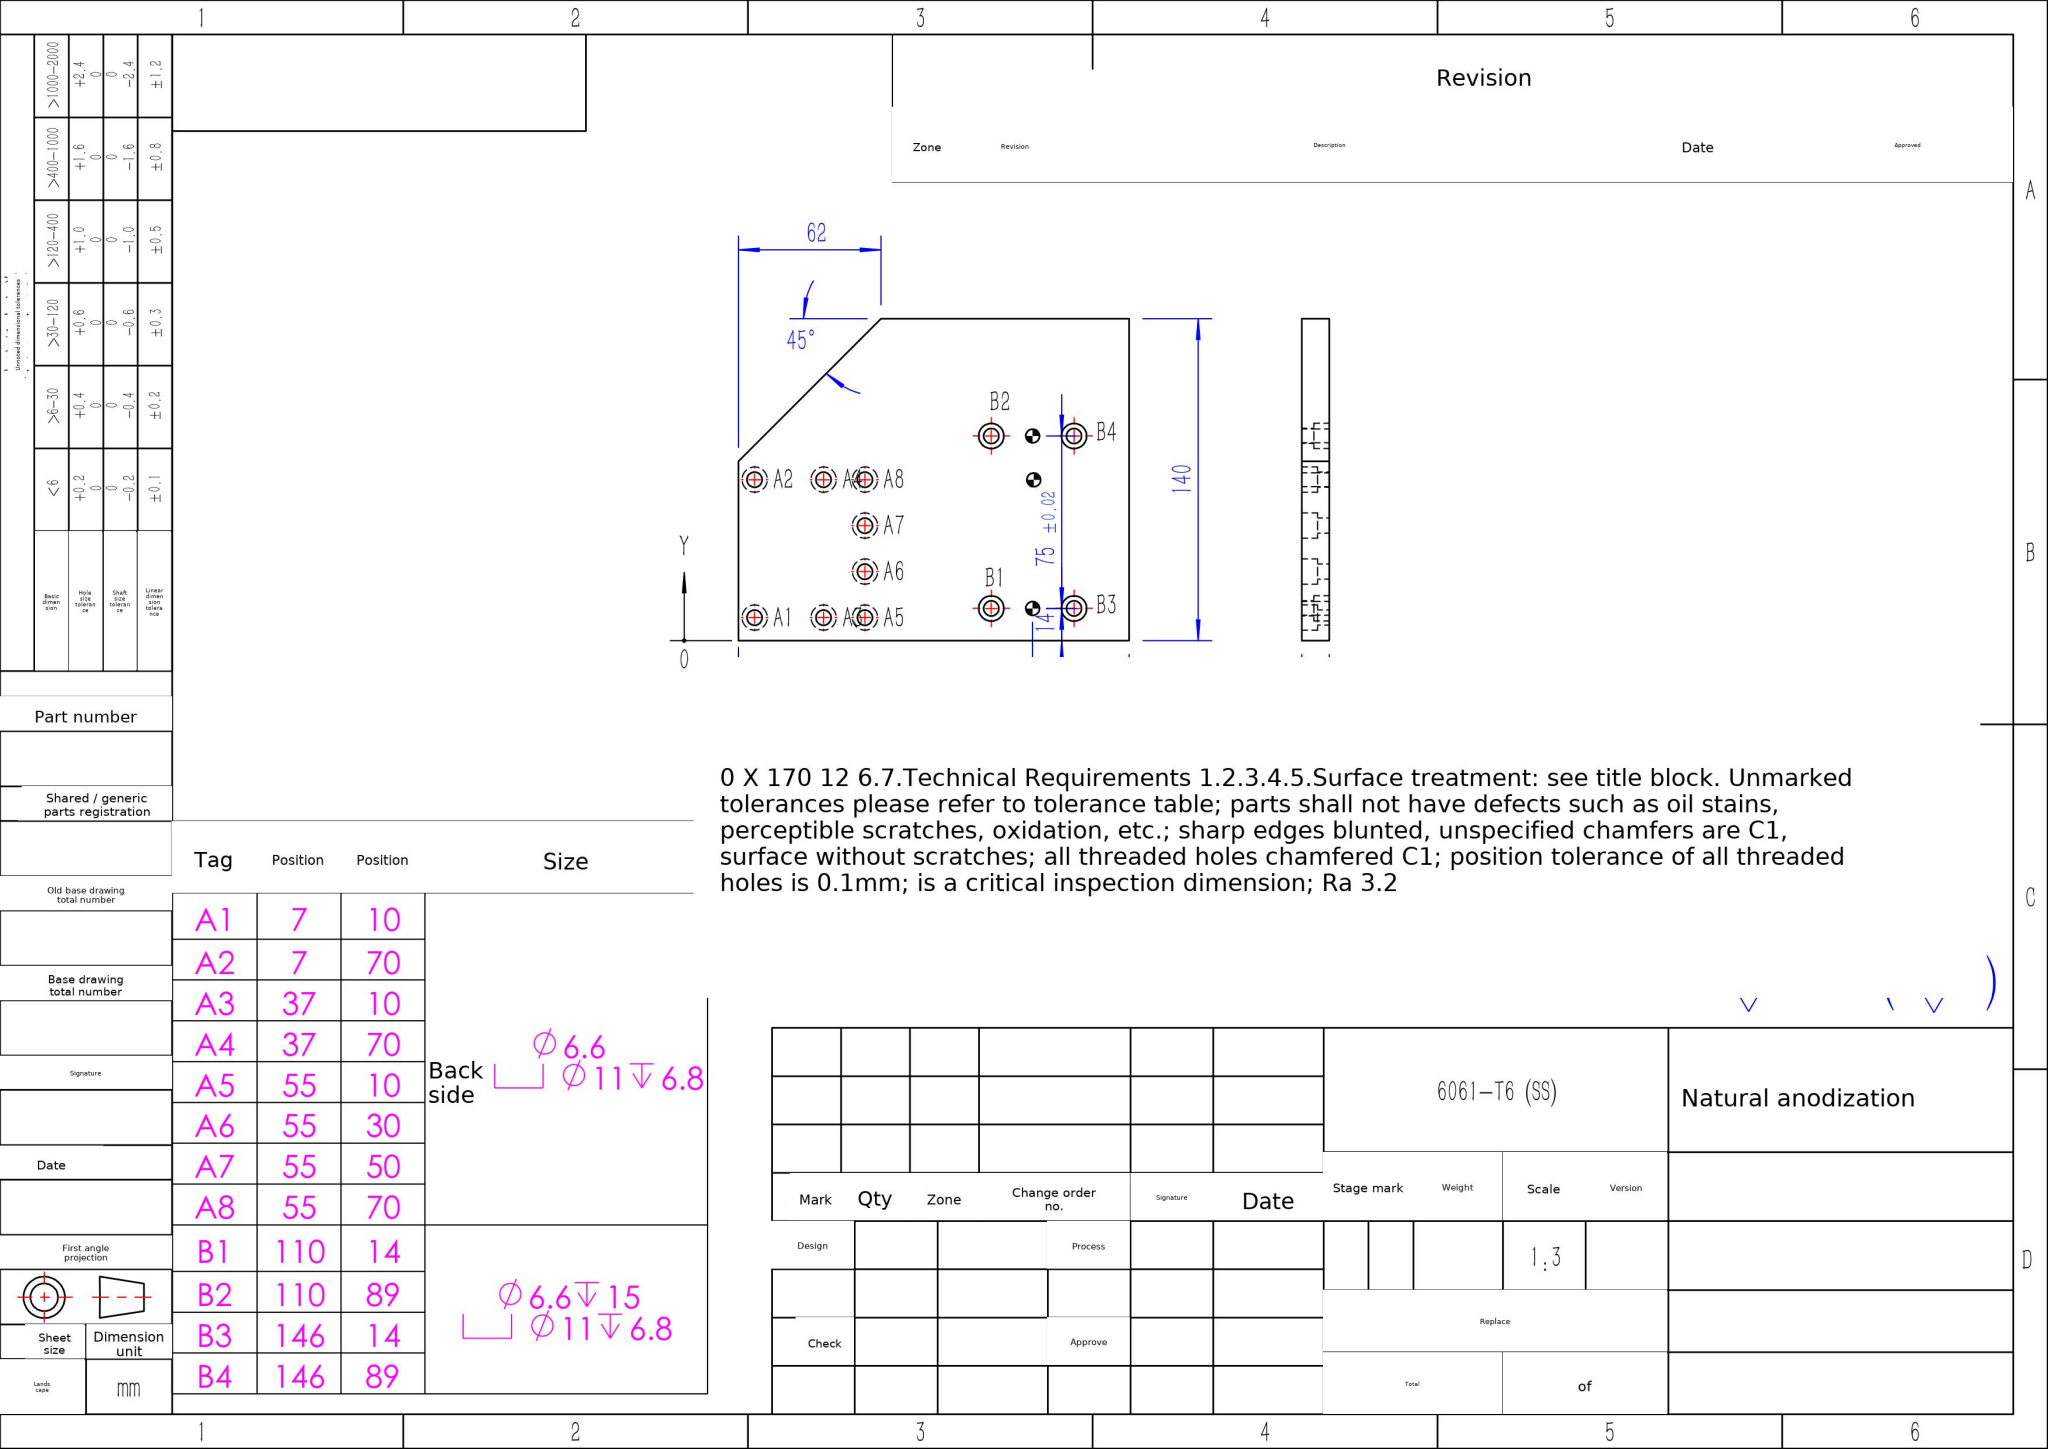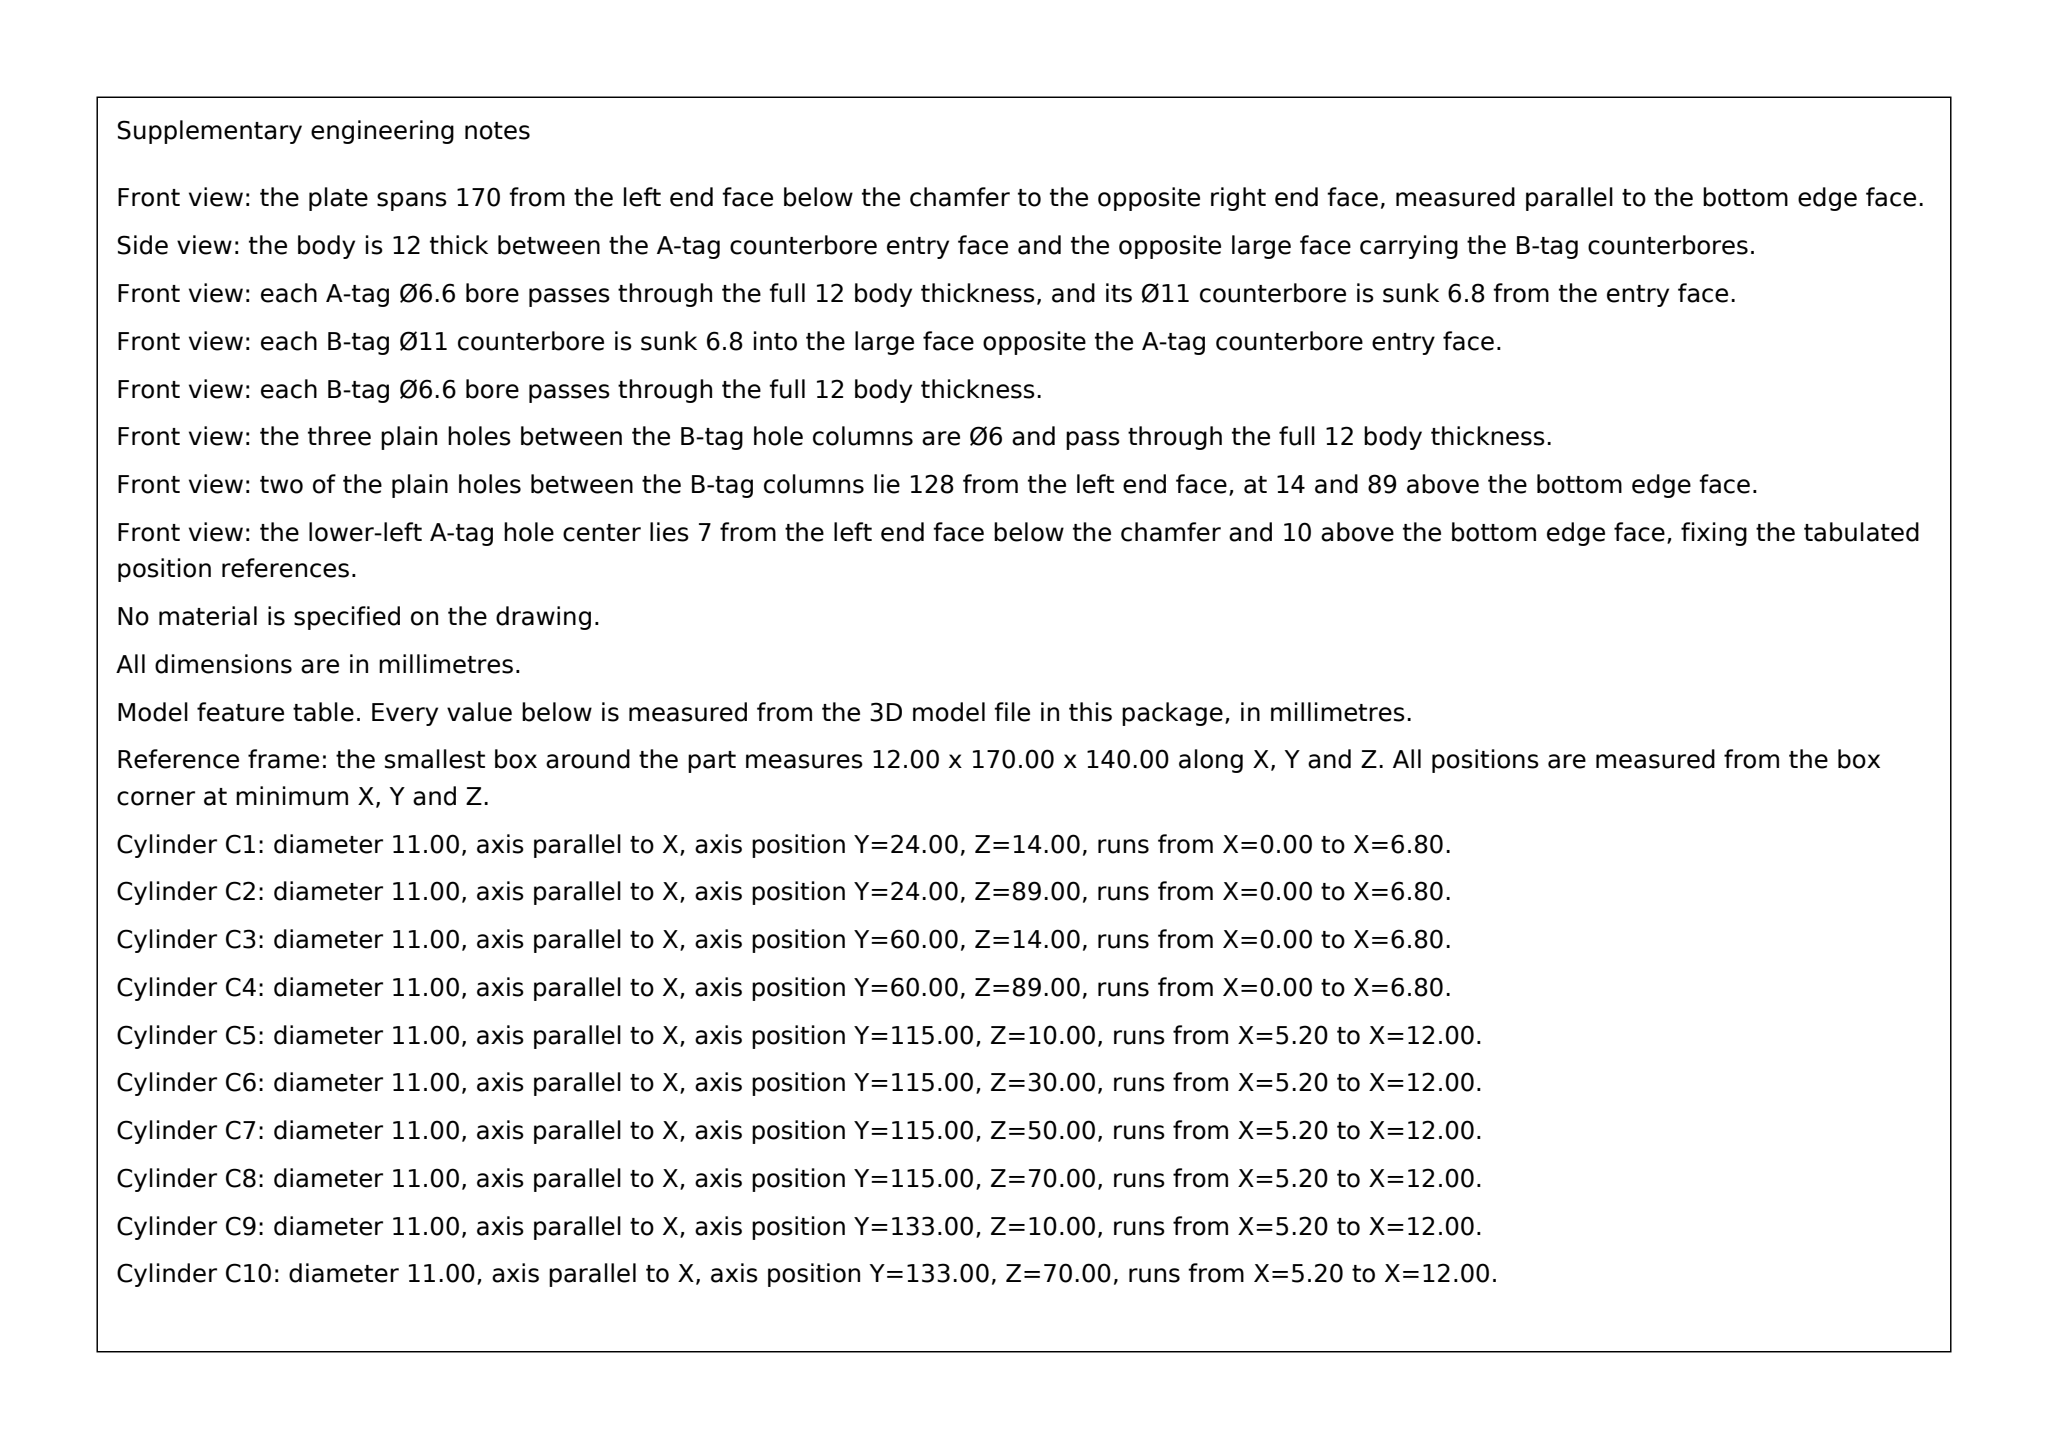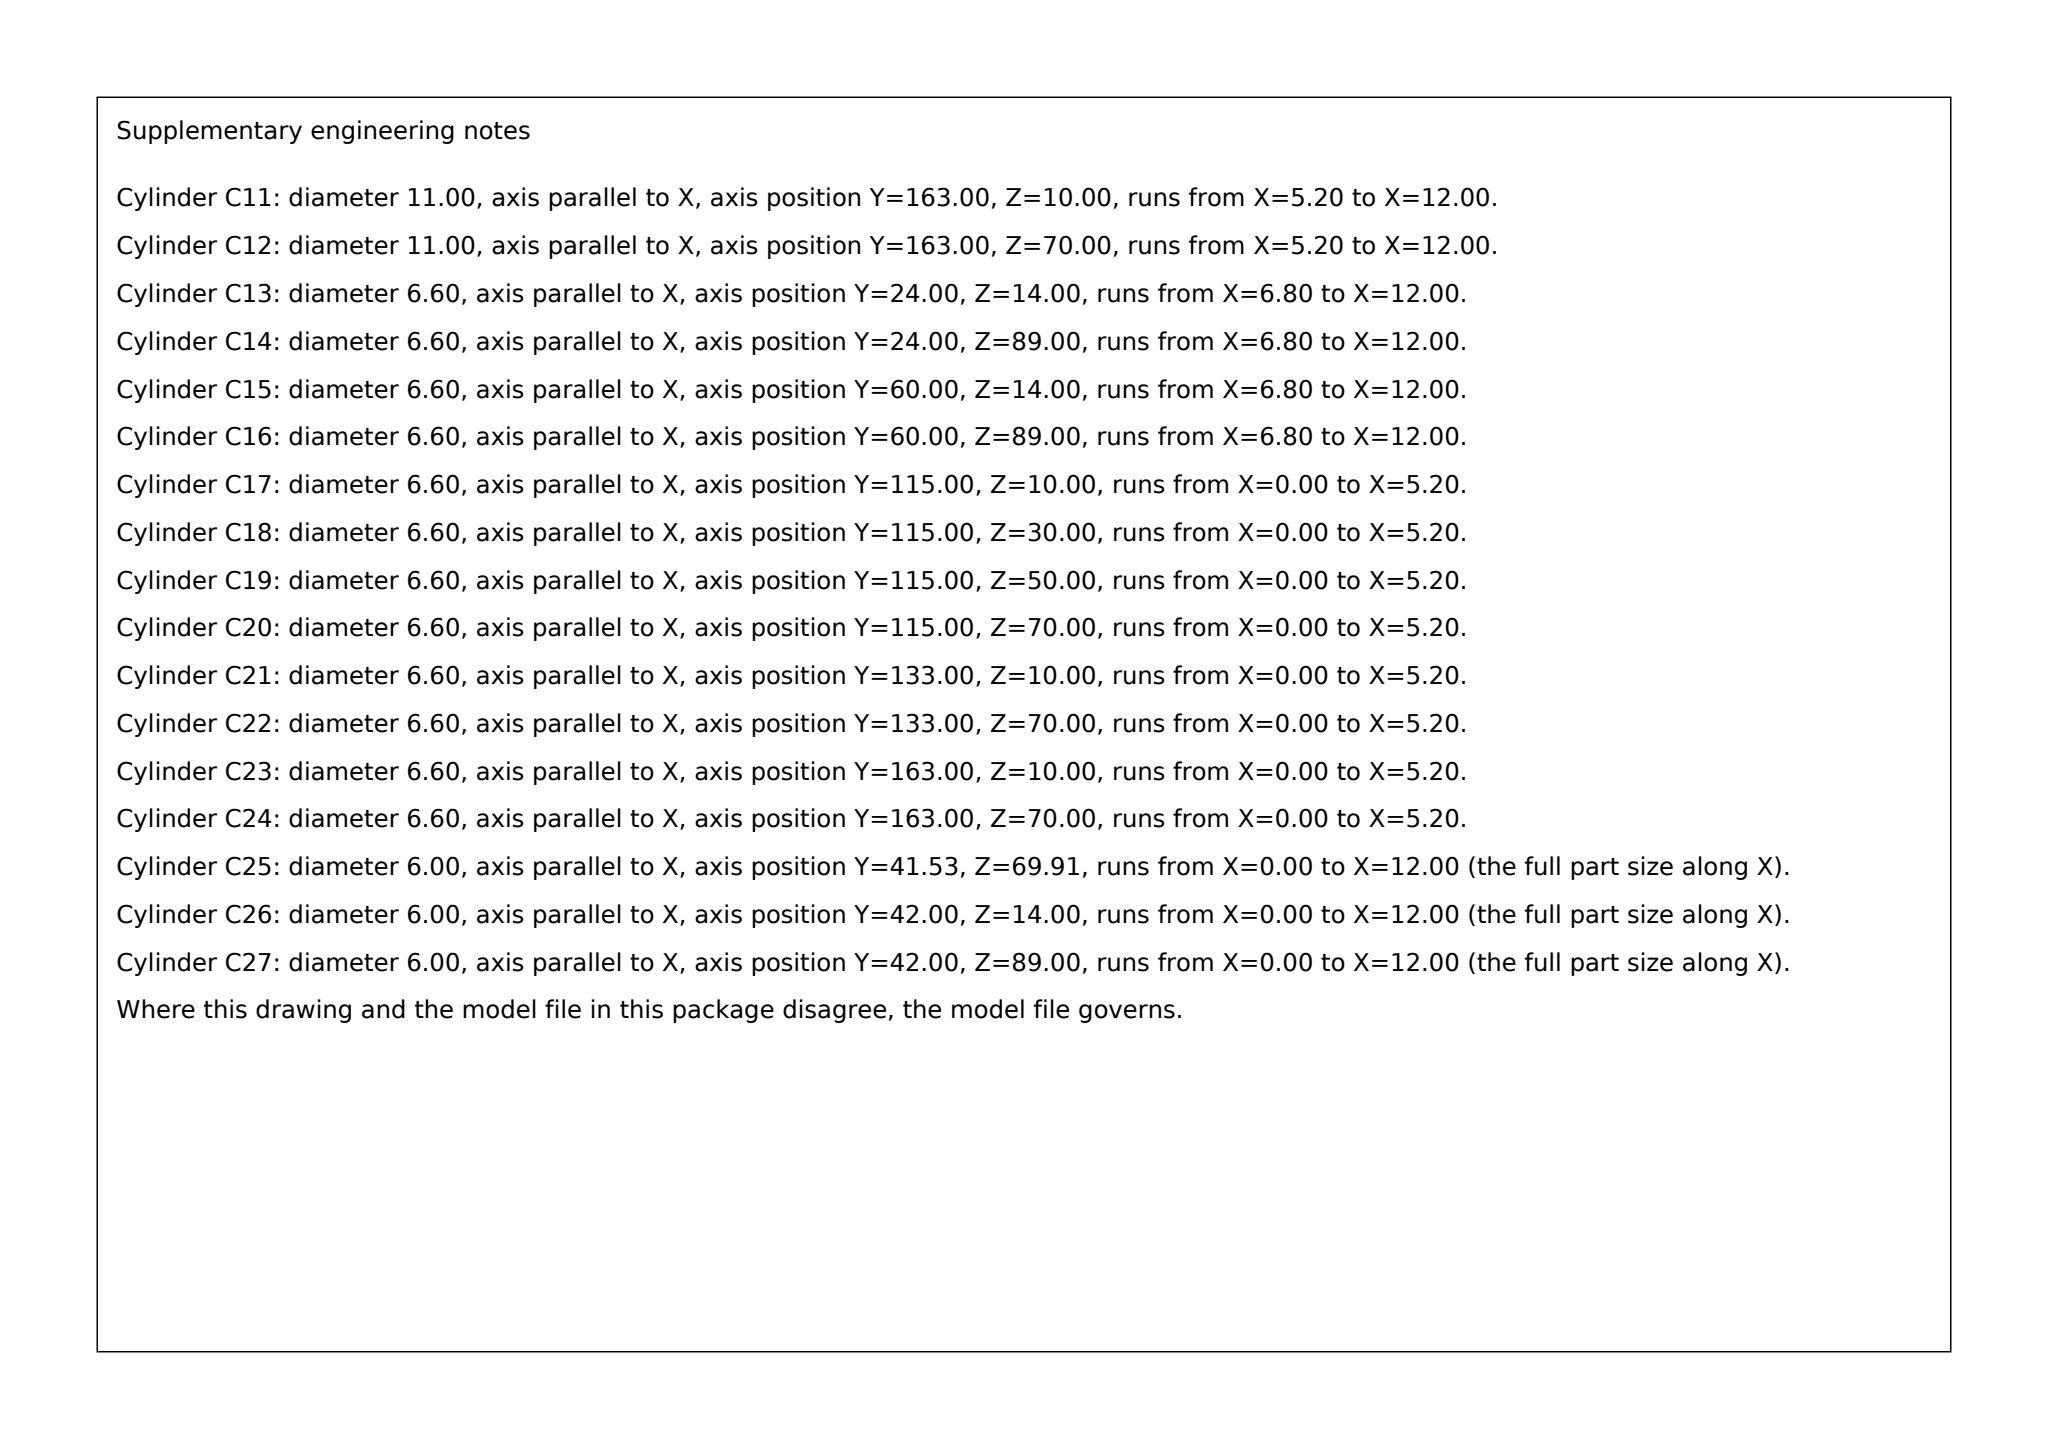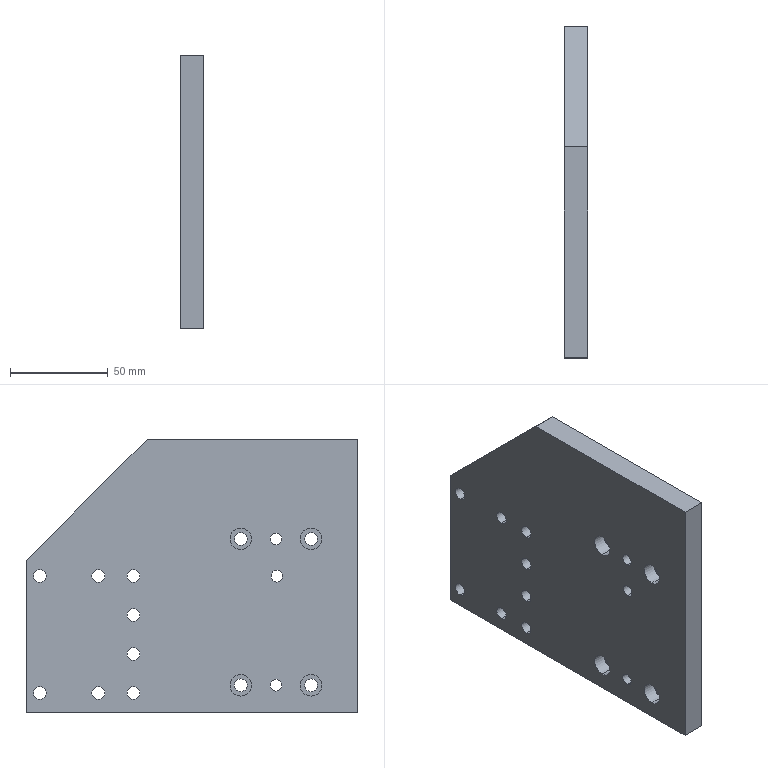Part | SolidWorks | mm | 1 solid | 73 faces | box 12 x 170 x 140 mm | volume 251629 mm3 | cylinder 54 | plane 19 | commonest cylinder face diameters 11 x24 6.6 x24 6 x6
Drawing notes:
Overall plate length 170 mm (long direction), full height 140 mm as shown. | from the solid: bbox_xyz [12.0, 170.0, 140.0]
Plate thickness 12 mm (side view) - between faces at x=0 and x=12. | from the solid: bbox_xyz x=12.0; axis_planes x 0.0 and x 12.0
3X Ø6 THRU (12 mm): at X128/Y14, X128/Y89 and X128.47/Y69.91 in the same X/Y datum system used by the A/B hole table. | from the solid: cylinders dia 6.0 axis x at [42.0,14.0], [42.0,89.0], [41.53,69.91], length 12.0 (170-42=128, 170-41.53=128.47)
B1-B4 (X110/Y14, X110/Y89, X146/Y14, X146/Y89): 4X Ø6.6 THRU, C'BORE Ø11 DP 6.8 from the front face (opposite the A-hole counterbore face). | from the solid: cylinders 6.6 L5.2 + 11.0 L6.8 at [24,14],[24,89],[60,14],[60,89] (5.2+6.8=12 thickness); axis_planes x=6.8 count 4
A1-A8: 8X Ø6.6 THRU, C'BORE Ø11 DP 6.8 from back side as noted. | from the solid: cylinders 6.6 L5.2 + 11.0 L6.8 at y=115/133/163 (5.2+6.8=12); axis_planes x=5.2 count 8
build123d program:
from build123d import *

# Parameters (mm, degrees)
SKETCH3_W                                         = 140
SKETCH3_H                                         = 170
BOSS_EXTRUDE2_DEPTH                               = 12
HOLE_SIZE_ACCORDING_TO_HEXAGON_SOCKET_D           = 6.6
HOLE_SIZE_ACCORDING_TO_HEXAGON_SOCKET_DEPTH       = 15
HOLE_SIZE_ACCORDING_TO_HEXAGON_SOCKET_CBORE_D     = 11
HOLE_SIZE_ACCORDING_TO_HEXAGON_SOCKET_CBORE_DEPTH = 6.8
HOLE_SIZE_ACCORDING_TO_HEXAGON_SOCKET_TIP         = 1.983
SIZE_MM_DOWEL_PIN_HOLE2_D                         = 6
SIZE_MM_DOWEL_PIN_HOLE2_DEPTH                     = 15
SIZE_MM_DOWEL_PIN_HOLE2_TIP                       = 1.803
CHAMFER1_SIZE                                     = 62
HOLE_SIZE_ACCORDING_TO_HEXAGON_SO_2_D             = 6.6
HOLE_SIZE_ACCORDING_TO_HEXAGON_SO_2_DEPTH         = 15
HOLE_SIZE_ACCORDING_TO_HEXAGON_SO_2_CBORE_D       = 11
HOLE_SIZE_ACCORDING_TO_HEXAGON_SO_2_CBORE_DEPTH   = 6.8
HOLE_SIZE_ACCORDING_TO_HEXAGON_SO_2_TIP           = 1.983
HOLE_SIZE_ACCORDING_TO_HEXAGON_SO_3_D             = 6.6
HOLE_SIZE_ACCORDING_TO_HEXAGON_SO_3_DEPTH         = 15
HOLE_SIZE_ACCORDING_TO_HEXAGON_SO_3_CBORE_D       = 11
HOLE_SIZE_ACCORDING_TO_HEXAGON_SO_3_CBORE_DEPTH   = 6.8
HOLE_SIZE_ACCORDING_TO_HEXAGON_SO_3_TIP           = 1.983


with BuildPart() as part:
    # Sketch3 → Boss-Extrude2 (new body)
    with BuildSketch(Plane(origin=(0, 0, 0), x_dir=(0, 0, -1), z_dir=(1, 0, 0))):
        with Locations((-30, -25)):
            Rectangle(SKETCH3_W, SKETCH3_H)
    extrude(amount=BOSS_EXTRUDE2_DEPTH)

    # Hole Size _ according to_ Hexagon Socket
    with Locations(Plane.ZY):
        with Locations((-26, -86), (-26, -50), (49, -86), (49, -50)):
            CounterBoreHole(HOLE_SIZE_ACCORDING_TO_HEXAGON_SOCKET_D / 2, HOLE_SIZE_ACCORDING_TO_HEXAGON_SOCKET_CBORE_D / 2, HOLE_SIZE_ACCORDING_TO_HEXAGON_SOCKET_CBORE_DEPTH, depth=HOLE_SIZE_ACCORDING_TO_HEXAGON_SOCKET_DEPTH)
            with Locations((0, 0, -(HOLE_SIZE_ACCORDING_TO_HEXAGON_SOCKET_DEPTH + HOLE_SIZE_ACCORDING_TO_HEXAGON_SOCKET_TIP / 2))):  # 118° drill point
                Cone(0, HOLE_SIZE_ACCORDING_TO_HEXAGON_SOCKET_D / 2, HOLE_SIZE_ACCORDING_TO_HEXAGON_SOCKET_TIP, mode=Mode.SUBTRACT)

    # Size mm Dowel Pin Hole2
    with Locations(Plane.ZY):
        with Locations((-26, -68), (29.913, -68.47), (49, -68)):
            Hole(SIZE_MM_DOWEL_PIN_HOLE2_D / 2, depth=SIZE_MM_DOWEL_PIN_HOLE2_DEPTH)
            with Locations((0, 0, -(SIZE_MM_DOWEL_PIN_HOLE2_DEPTH + SIZE_MM_DOWEL_PIN_HOLE2_TIP / 2))):  # 118° drill point
                Cone(0, SIZE_MM_DOWEL_PIN_HOLE2_D / 2, SIZE_MM_DOWEL_PIN_HOLE2_TIP, mode=Mode.SUBTRACT)

    # Chamfer1
    chamfer1_edges = [part.edges().sort_by_distance(p)[0] for p in [
        (6, 60, 100),
    ]]
    chamfer(chamfer1_edges, length=CHAMFER1_SIZE)

    # Hole Size _ according to_ Hexagon So 2
    with Locations(Plane(origin=(12, 0, 0), x_dir=(0, 0, -1), z_dir=(1, 0, 0))):
        with Locations((30, 5), (10, 5), (-10, 5), (-30, 5)):
            CounterBoreHole(HOLE_SIZE_ACCORDING_TO_HEXAGON_SO_2_D / 2, HOLE_SIZE_ACCORDING_TO_HEXAGON_SO_2_CBORE_D / 2, HOLE_SIZE_ACCORDING_TO_HEXAGON_SO_2_CBORE_DEPTH, depth=HOLE_SIZE_ACCORDING_TO_HEXAGON_SO_2_DEPTH)
            with Locations((0, 0, -(HOLE_SIZE_ACCORDING_TO_HEXAGON_SO_2_DEPTH + HOLE_SIZE_ACCORDING_TO_HEXAGON_SO_2_TIP / 2))):  # 118° drill point
                Cone(0, HOLE_SIZE_ACCORDING_TO_HEXAGON_SO_2_D / 2, HOLE_SIZE_ACCORDING_TO_HEXAGON_SO_2_TIP, mode=Mode.SUBTRACT)

    # Hole Size _ according to_ Hexagon So 3
    with Locations(Plane(origin=(12, 0, 0), x_dir=(0, 0, -1), z_dir=(1, 0, 0))):
        with Locations((-30, 23), (-30, 53), (30, 53), (30, 23)):
            CounterBoreHole(HOLE_SIZE_ACCORDING_TO_HEXAGON_SO_3_D / 2, HOLE_SIZE_ACCORDING_TO_HEXAGON_SO_3_CBORE_D / 2, HOLE_SIZE_ACCORDING_TO_HEXAGON_SO_3_CBORE_DEPTH, depth=HOLE_SIZE_ACCORDING_TO_HEXAGON_SO_3_DEPTH)
            with Locations((0, 0, -(HOLE_SIZE_ACCORDING_TO_HEXAGON_SO_3_DEPTH + HOLE_SIZE_ACCORDING_TO_HEXAGON_SO_3_TIP / 2))):  # 118° drill point
                Cone(0, HOLE_SIZE_ACCORDING_TO_HEXAGON_SO_3_D / 2, HOLE_SIZE_ACCORDING_TO_HEXAGON_SO_3_TIP, mode=Mode.SUBTRACT)


solid = part.part